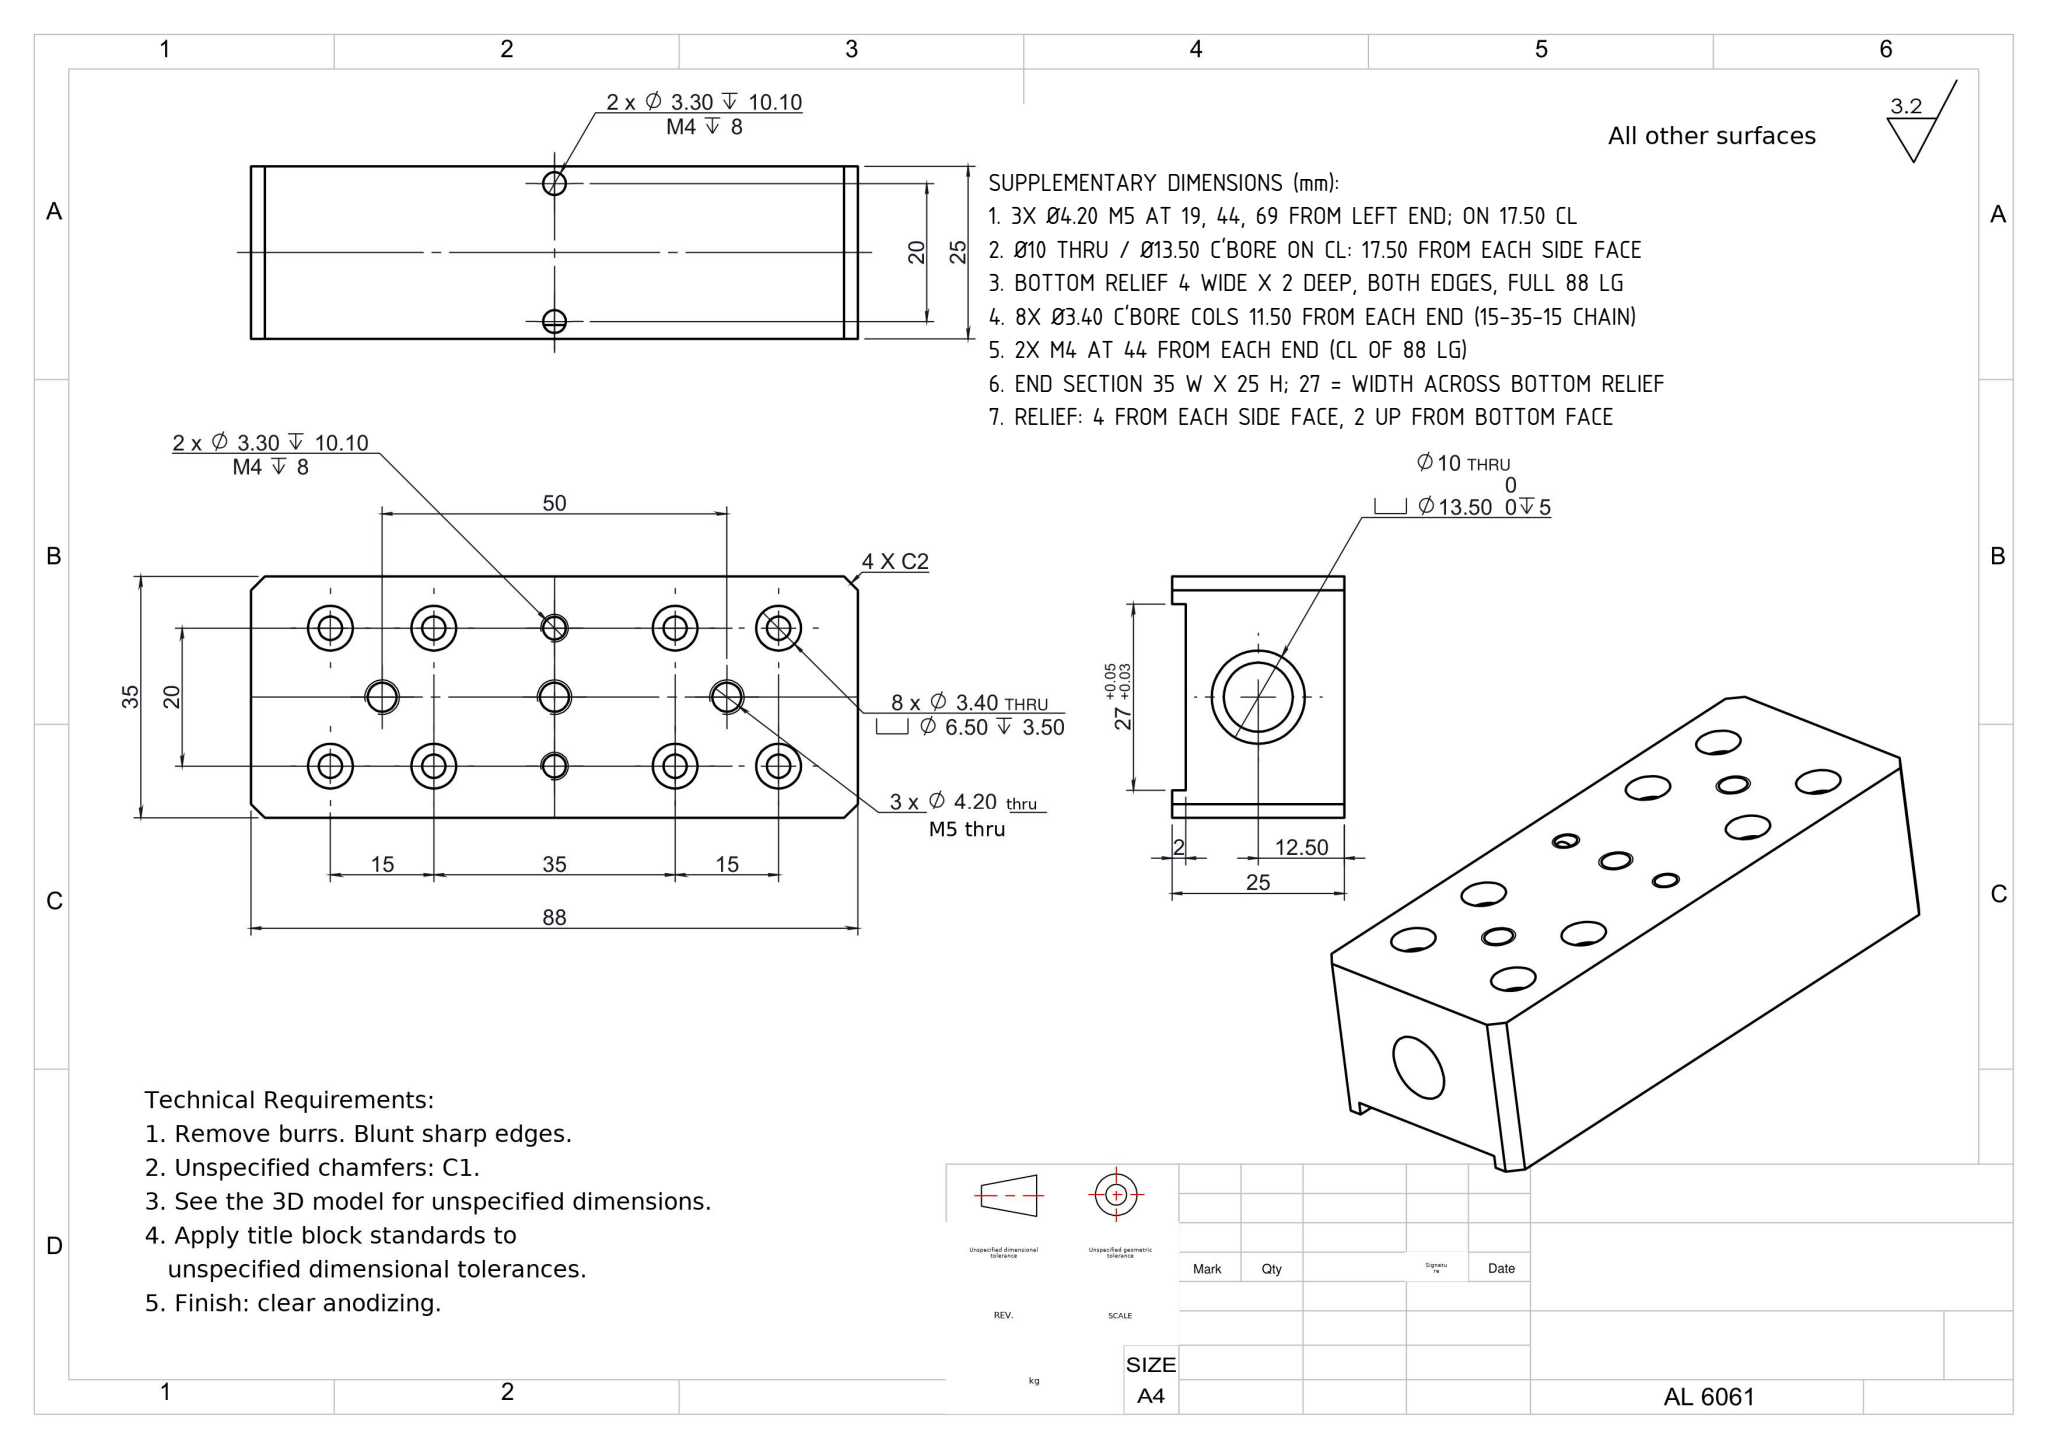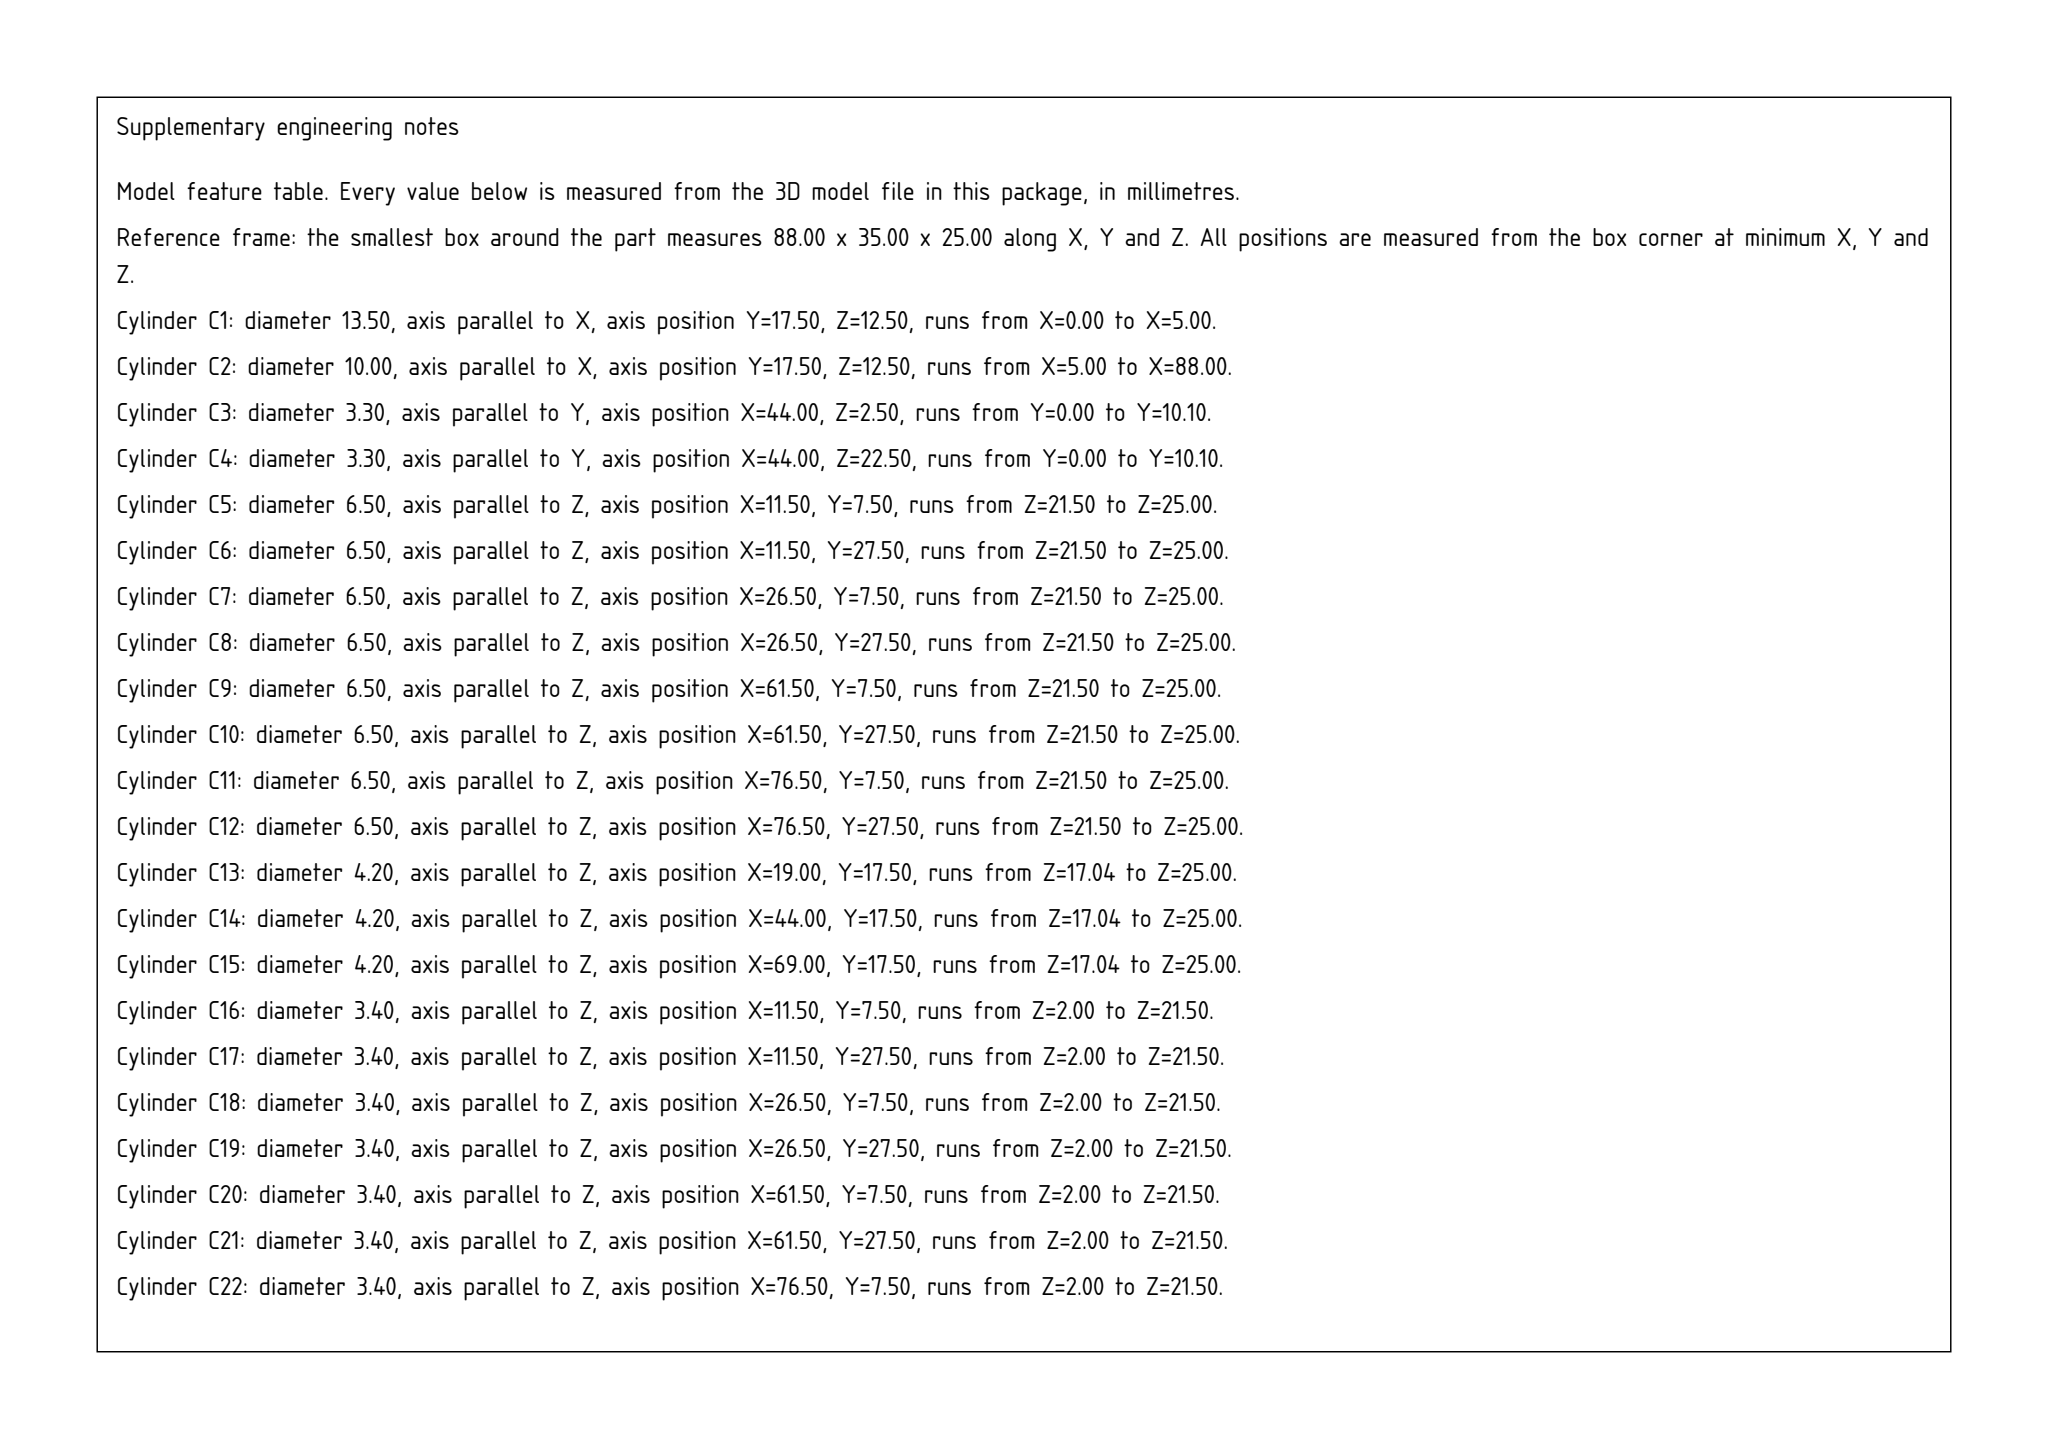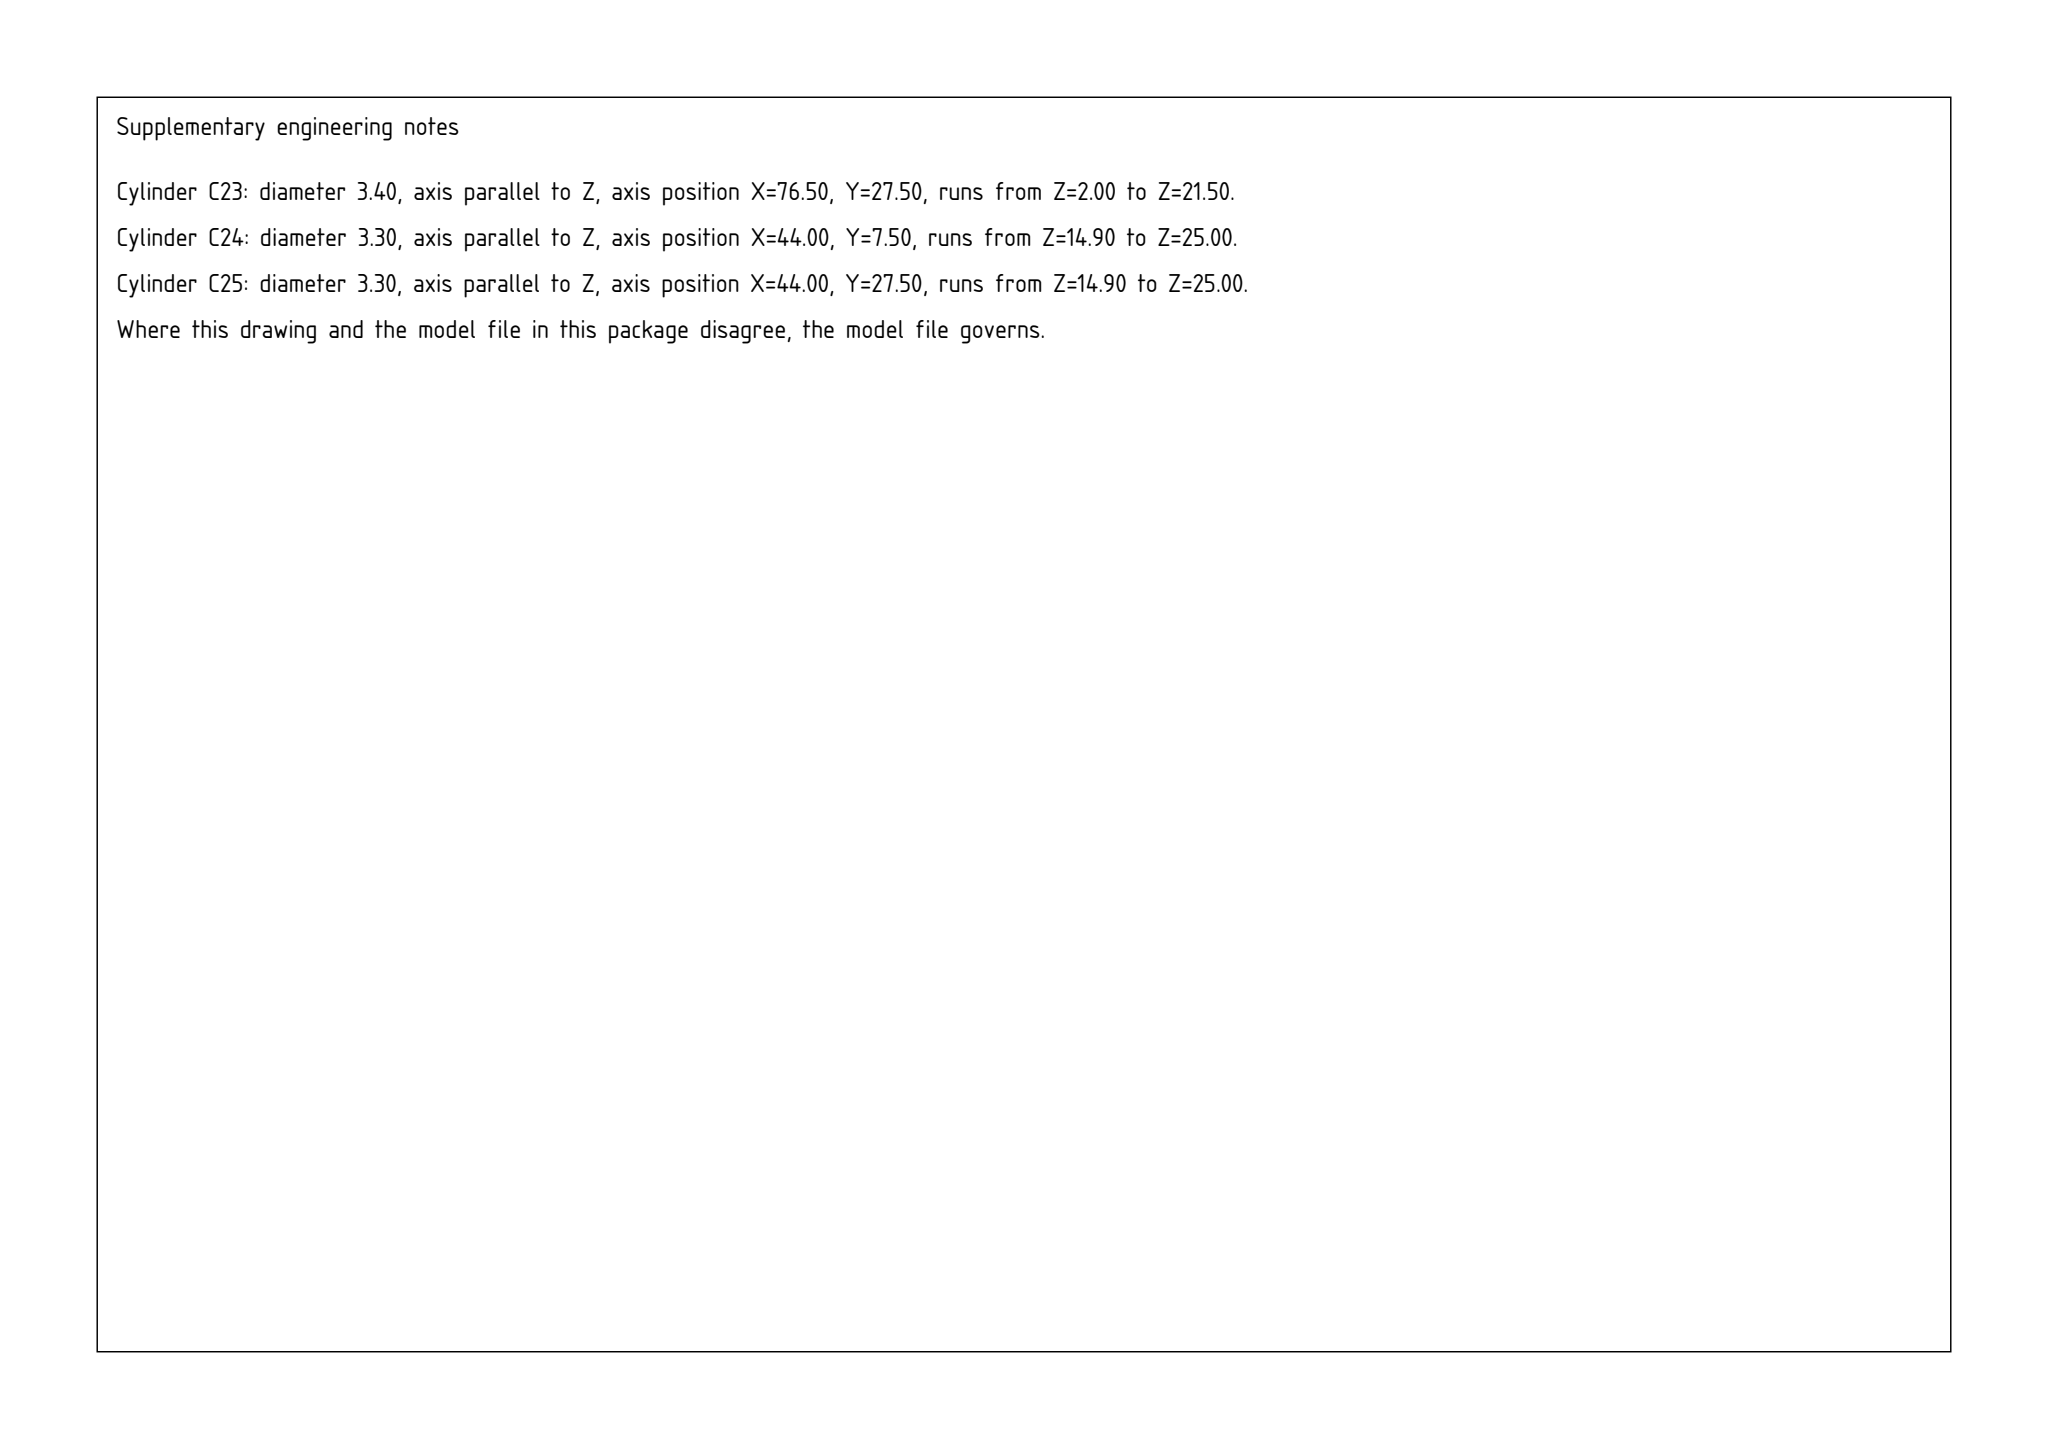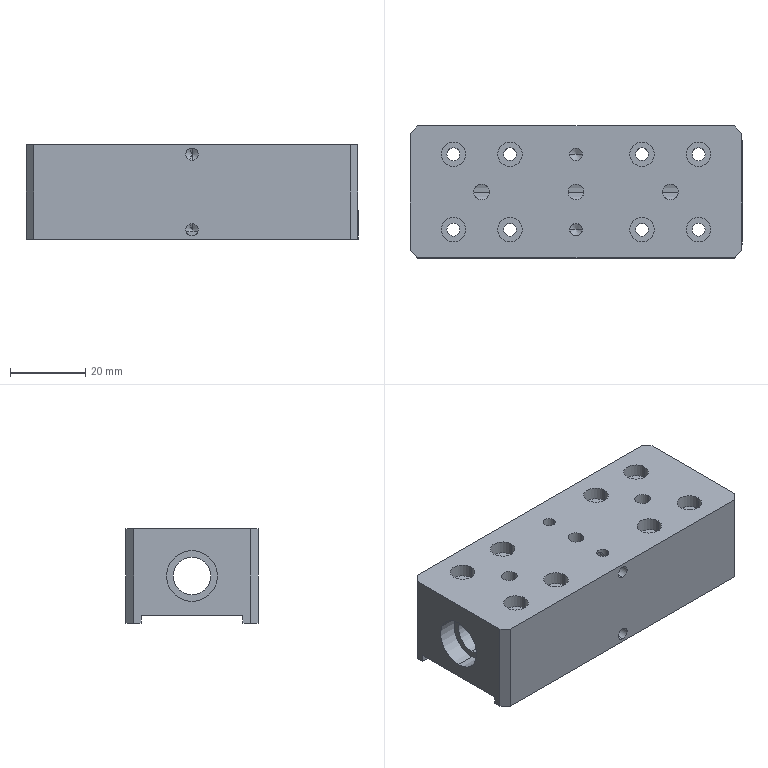Part | SolidWorks | mm | 1 solid | 85 faces | box 88 x 35 x 25 mm | volume 61836 mm3 | cylinder 54 | plane 23 | cone 8 | commonest cylinder face diameters 6.5 x16 3.4 x16 3.3 x12 4.2 x6 13.5 x2 10 x2
build123d program:
from build123d import *

# Parameters (mm, degrees)
SKETCH1_W                                       = 88
SKETCH1_H                                       = 35
BOSS_EXTRUDE1_DEPTH                             = 12.5
SKETCH2_R                                       = 5
CUT_EXTRUDE1_DEPTH                              = 91.59
M5_TAPPED_HOLE1_REACH                           = 55.547
M5_TAPPED_HOLE1_BORE_R                          = 2.1
SKETCH9_W                                       = 88
SKETCH9_H                                       = 27
CUT_EXTRUDE2_DEPTH                              = 2
SKETCH11_R                                      = 6.75
CUT_EXTRUDE3_DEPTH                              = 5
M3_HEX_SOCKET_HEAD_CAP_SCREW_CBORE1_D           = 3.4
M3_HEX_SOCKET_HEAD_CAP_SCREW_CBORE1_CBORE_D     = 6.5
M3_HEX_SOCKET_HEAD_CAP_SCREW_CBORE1_CBORE_DEPTH = 3.5
M4_TAPPED_HOLE1_D                               = 3.3
M4_TAPPED_HOLE1_DEPTH                           = 10.1
M4_TAPPED_HOLE1_TIP                             = 0.9914
CHAMFER1_SIZE                                   = 2
M4_TAPPED_HOLE2_D                               = 3.3
M4_TAPPED_HOLE2_DEPTH                           = 10.1
M4_TAPPED_HOLE2_TIP                             = 0.9914


with BuildPart() as part:
    # Sketch1 → Boss-Extrude1 (new, symmetric)
    with BuildSketch(Plane.XY):
        Rectangle(SKETCH1_W, SKETCH1_H)
    extrude(amount=BOSS_EXTRUDE1_DEPTH, both=True)

    # Sketch2 → Cut-Extrude1 (cut, through all)
    with BuildSketch(Plane.ZY.offset(44)):
        Circle(SKETCH2_R)
    extrude(amount=-CUT_EXTRUDE1_DEPTH, mode=Mode.SUBTRACT)

    # M5 Tapped Hole1 bore → M5 Tapped Hole1 (cut, up to next)
    with BuildSketch(Plane.XY.offset(12.5), mode=Mode.PRIVATE) as m5_tapped_hole1_sk1:
        with Locations((-25, 0)):
            Circle(M5_TAPPED_HOLE1_BORE_R)
    m5_tapped_hole1_tool1 = extrude(m5_tapped_hole1_sk1.sketch, amount=-M5_TAPPED_HOLE1_REACH, mode=Mode.PRIVATE) & part.part
    # M5 Tapped Hole1 bore → M5 Tapped Hole1 (cut, up to next)
    with BuildSketch(Plane.XY.offset(12.5), mode=Mode.PRIVATE) as m5_tapped_hole1_sk2:
        Circle(M5_TAPPED_HOLE1_BORE_R)
    m5_tapped_hole1_tool2 = extrude(m5_tapped_hole1_sk2.sketch, amount=-M5_TAPPED_HOLE1_REACH, mode=Mode.PRIVATE) & part.part
    # M5 Tapped Hole1 bore → M5 Tapped Hole1 (cut, up to next)
    with BuildSketch(Plane.XY.offset(12.5), mode=Mode.PRIVATE) as m5_tapped_hole1_sk3:
        with Locations((25, 0)):
            Circle(M5_TAPPED_HOLE1_BORE_R)
    m5_tapped_hole1_tool3 = extrude(m5_tapped_hole1_sk3.sketch, amount=-M5_TAPPED_HOLE1_REACH, mode=Mode.PRIVATE) & part.part
    add(m5_tapped_hole1_tool1.solids().sort_by_distance((-25, 0, 12.5))[0], mode=Mode.SUBTRACT)
    add(m5_tapped_hole1_tool2.solids().sort_by_distance((0, 0, 12.5))[0], mode=Mode.SUBTRACT)
    add(m5_tapped_hole1_tool3.solids().sort_by_distance((25, 0, 12.5))[0], mode=Mode.SUBTRACT)

    # Sketch9 → Cut-Extrude2 (cut)
    with BuildSketch(Plane(origin=(0, 0, -12.5), x_dir=(-1, 0, 0), z_dir=(0, 0, -1))):
        Rectangle(SKETCH9_W, SKETCH9_H)
    extrude(amount=-CUT_EXTRUDE2_DEPTH, mode=Mode.SUBTRACT)

    # Sketch11 → Cut-Extrude3 (cut)
    with BuildSketch(Plane.ZY.offset(44)):
        Circle(SKETCH11_R)
    extrude(amount=-CUT_EXTRUDE3_DEPTH, mode=Mode.SUBTRACT)

    # M3 Hex Socket Head Cap Screw CBORE1 (through all)
    with Locations(Plane.XY.offset(12.5)):
        with Locations((32.5, 10), (17.5, 10), (32.5, -10), (17.5, -10)):
            m3_hex_socket_head_cap_screw_cbore1 = CounterBoreHole(M3_HEX_SOCKET_HEAD_CAP_SCREW_CBORE1_D / 2, M3_HEX_SOCKET_HEAD_CAP_SCREW_CBORE1_CBORE_D / 2, M3_HEX_SOCKET_HEAD_CAP_SCREW_CBORE1_CBORE_DEPTH)

    # Mirror1: M3 Hex Socket Head Cap Screw CBORE1 across plane
    add(m3_hex_socket_head_cap_screw_cbore1.mirror(Plane(origin=(0, 0, 0), x_dir=(0, 0, 1), z_dir=(1, 0, 0))), mode=Mode.SUBTRACT)

    # M4 Tapped Hole1
    with Locations(Plane.XY.offset(12.5)):
        with Locations((0, 10), (0, -10)):
            Hole(M4_TAPPED_HOLE1_D / 2, depth=M4_TAPPED_HOLE1_DEPTH)
            with Locations((0, 0, -(M4_TAPPED_HOLE1_DEPTH + M4_TAPPED_HOLE1_TIP / 2))):  # 118° drill point
                Cone(0, M4_TAPPED_HOLE1_D / 2, M4_TAPPED_HOLE1_TIP, mode=Mode.SUBTRACT)

    # Chamfer1
    chamfer1_edges = [part.edges().sort_by_distance(p)[0] for p in [
        (44, -17.5, 0),
        (-44, -17.5, 0),
        (-44, 17.5, 0),
        (44, 17.5, 0),
    ]]
    chamfer(chamfer1_edges, length=CHAMFER1_SIZE)

    # M4 Tapped Hole2
    with Locations(Plane(origin=(0, -17.5, 0), x_dir=(-1, 0, 0), z_dir=(0, -1, 0))):
        with Locations((0, -10), (0, 10)):
            Hole(M4_TAPPED_HOLE2_D / 2, depth=M4_TAPPED_HOLE2_DEPTH)
            with Locations((0, 0, -(M4_TAPPED_HOLE2_DEPTH + M4_TAPPED_HOLE2_TIP / 2))):  # 118° drill point
                Cone(0, M4_TAPPED_HOLE2_D / 2, M4_TAPPED_HOLE2_TIP, mode=Mode.SUBTRACT)


solid = part.part